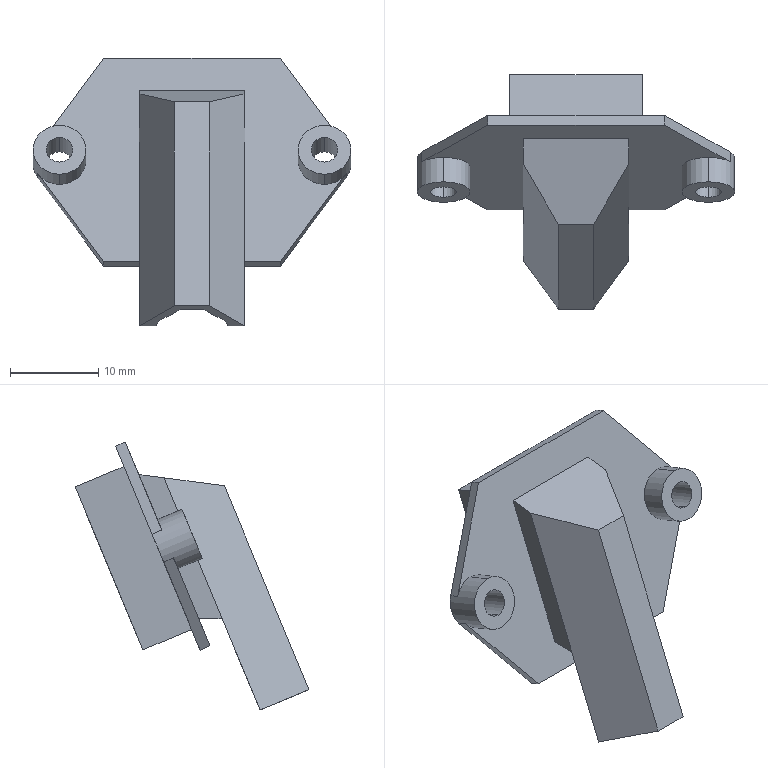Component | SolidWorks | SeedingAssemblyA-1_SeedingSlot-10 | 1 solid | 58 faces | volume 1853 mm3 | plane 48 | cylinder 10 | commonest cylinder face diameters 3 x4 6 x4 8.1 x2